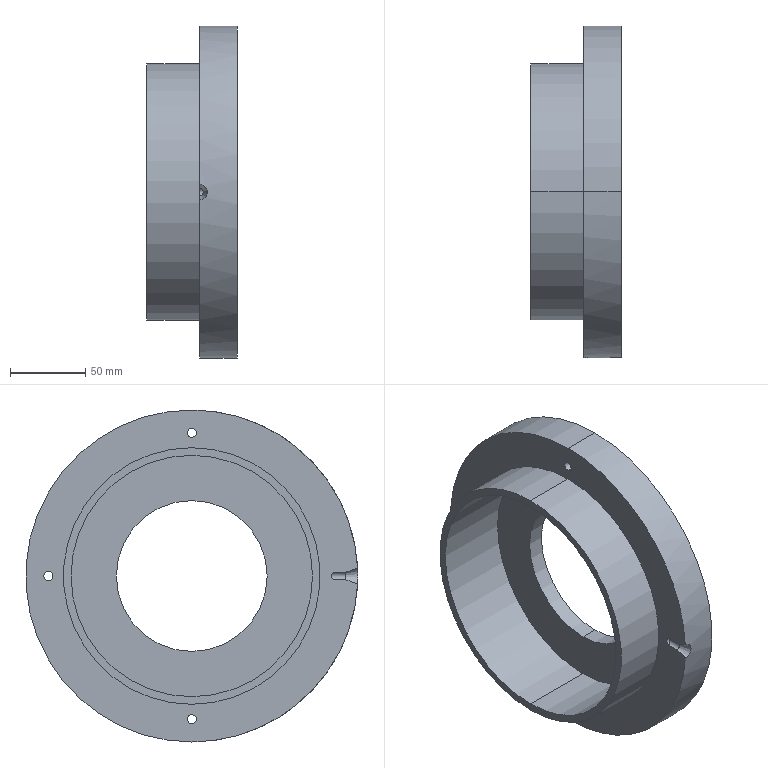Component | SolidWorks | EndCap-1 | 1 solid | 27 faces | box 60 x 220 x 220 mm | volume 670749 mm3 | cylinder 16 | cone 7 | plane 4 | commonest cylinder face diameters 6 x6 100 x2 160 x2 170 x2 220 x2 5 x2
STEP:
#1=COLOUR_RGB('',0.7922,0.8196,0.9333);
#2=FILL_AREA_STYLE_COLOUR('',#1);
#3=FILL_AREA_STYLE('',(#2));
#4=SURFACE_STYLE_FILL_AREA(#3);
#5=SURFACE_SIDE_STYLE('',(#4));
#6=SURFACE_STYLE_USAGE(.BOTH.,#5);
#7=PRESENTATION_STYLE_ASSIGNMENT((#6));
#8=CARTESIAN_POINT('',(-0.01969,3.74,0.1181));
#9=VERTEX_POINT('',#8);
#10=CARTESIAN_POINT('',(-0.01969,3.74,-0.1181));
#11=VERTEX_POINT('',#10);
#12=CARTESIAN_POINT('',(-0.01969,3.74,-0.));
#13=DIRECTION('',(1.,0.,-0.));
#14=DIRECTION('',(0.,0.,1.));
#15=AXIS2_PLACEMENT_3D('',#12,#13,#14);
#16=CIRCLE('',#15,0.1181);
#17=EDGE_CURVE('',#9,#11,#16,.T.);
#18=ORIENTED_EDGE('',*,*,#17,.F.);
#19=CARTESIAN_POINT('',(-0.,3.74,0.1378));
#20=VERTEX_POINT('',#19);
#21=CARTESIAN_POINT('',(-0.,3.74,0.1378));
#22=DIRECTION('',(0.7071,0.,0.7071));
#23=VECTOR('',#22,39.37);
#24=LINE('',#21,#23);
#25=EDGE_CURVE('',#9,#20,#24,.T.);
#26=ORIENTED_EDGE('',*,*,#25,.T.);
#27=CARTESIAN_POINT('',(-0.,3.74,-0.1378));
#28=VERTEX_POINT('',#27);
#29=CARTESIAN_POINT('',(-0.,3.74,-0.));
#30=DIRECTION('',(-1.,-0.,0.));
#31=DIRECTION('',(0.,0.,1.));
#32=AXIS2_PLACEMENT_3D('',#29,#30,#31);
#33=CIRCLE('',#32,0.1378);
#34=EDGE_CURVE('',#28,#20,#33,.T.);
#35=ORIENTED_EDGE('',*,*,#34,.F.);
#36=CARTESIAN_POINT('',(-0.,3.74,-0.1378));
#37=DIRECTION('',(0.7071,0.,-0.7071));
#38=VECTOR('',#37,39.37);
#39=LINE('',#36,#38);
#40=EDGE_CURVE('',#11,#28,#39,.T.);
#41=ORIENTED_EDGE('',*,*,#40,.F.);
#42=EDGE_LOOP('',(#18,#26,#35,#41));
#43=FACE_OUTER_BOUND('',#42,.T.);
#44=CARTESIAN_POINT('',(-0.,3.74,-0.));
#45=DIRECTION('',(1.,0.,-0.));
#46=DIRECTION('',(-0.,0.,-1.));
#47=AXIS2_PLACEMENT_3D('',#44,#45,#46);
#48=CONICAL_SURFACE('',#47,0.1378,0.7854);
#49=ADVANCED_FACE('',(#43),#48,.F.);
#50=CARTESIAN_POINT('',(-0.01969,-0.,-3.622));
#51=VERTEX_POINT('',#50);
#52=CARTESIAN_POINT('',(-0.01969,-0.,-3.858));
#53=VERTEX_POINT('',#52);
#54=CARTESIAN_POINT('',(-0.01969,-0.,-3.74));
#55=DIRECTION('',(1.,0.,-0.));
#56=DIRECTION('',(0.,0.,1.));
#57=AXIS2_PLACEMENT_3D('',#54,#55,#56);
#58=CIRCLE('',#57,0.1181);
#59=EDGE_CURVE('',#51,#53,#58,.T.);
#60=ORIENTED_EDGE('',*,*,#59,.F.);
#61=CARTESIAN_POINT('',(-0.,0.,-3.602));
#62=VERTEX_POINT('',#61);
#63=CARTESIAN_POINT('',(-0.,0.,-3.602));
#64=DIRECTION('',(0.7071,0.,0.7071));
#65=VECTOR('',#64,39.37);
#66=LINE('',#63,#65);
#67=EDGE_CURVE('',#51,#62,#66,.T.);
#68=ORIENTED_EDGE('',*,*,#67,.T.);
#69=CARTESIAN_POINT('',(-0.,0.,-3.878));
#70=VERTEX_POINT('',#69);
#71=CARTESIAN_POINT('',(-0.,0.,-3.74));
#72=DIRECTION('',(-1.,-0.,0.));
#73=DIRECTION('',(0.,0.,1.));
#74=AXIS2_PLACEMENT_3D('',#71,#72,#73);
#75=CIRCLE('',#74,0.1378);
#76=EDGE_CURVE('',#70,#62,#75,.T.);
#77=ORIENTED_EDGE('',*,*,#76,.F.);
#78=CARTESIAN_POINT('',(-0.,0.,-3.878));
#79=DIRECTION('',(0.7071,0.,-0.7071));
#80=VECTOR('',#79,39.37);
#81=LINE('',#78,#80);
#82=EDGE_CURVE('',#53,#70,#81,.T.);
#83=ORIENTED_EDGE('',*,*,#82,.F.);
#84=EDGE_LOOP('',(#60,#68,#77,#83));
#85=FACE_OUTER_BOUND('',#84,.T.);
#86=CARTESIAN_POINT('',(-0.,0.,-3.74));
#87=DIRECTION('',(1.,0.,-0.));
#88=DIRECTION('',(-0.,0.,-1.));
#89=AXIS2_PLACEMENT_3D('',#86,#87,#88);
#90=CONICAL_SURFACE('',#89,0.1378,0.7854);
#91=ADVANCED_FACE('',(#85),#90,.F.);
#92=CARTESIAN_POINT('',(-0.01969,-0.,3.858));
#93=VERTEX_POINT('',#92);
#94=CARTESIAN_POINT('',(-0.01969,-0.,3.622));
#95=VERTEX_POINT('',#94);
#96=CARTESIAN_POINT('',(-0.01969,-0.,3.74));
#97=DIRECTION('',(1.,0.,-0.));
#98=DIRECTION('',(0.,0.,1.));
#99=AXIS2_PLACEMENT_3D('',#96,#97,#98);
#100=CIRCLE('',#99,0.1181);
#101=EDGE_CURVE('',#93,#95,#100,.T.);
#102=ORIENTED_EDGE('',*,*,#101,.F.);
#103=CARTESIAN_POINT('',(0.,0.,3.878));
#104=VERTEX_POINT('',#103);
#105=CARTESIAN_POINT('',(0.,0.,3.878));
#106=DIRECTION('',(0.7071,0.,0.7071));
#107=VECTOR('',#106,39.37);
#108=LINE('',#105,#107);
#109=EDGE_CURVE('',#93,#104,#108,.T.);
#110=ORIENTED_EDGE('',*,*,#109,.T.);
#111=CARTESIAN_POINT('',(0.,0.,3.602));
#112=VERTEX_POINT('',#111);
#113=CARTESIAN_POINT('',(0.,0.,3.74));
#114=DIRECTION('',(-1.,-0.,0.));
#115=DIRECTION('',(0.,0.,1.));
#116=AXIS2_PLACEMENT_3D('',#113,#114,#115);
#117=CIRCLE('',#116,0.1378);
#118=EDGE_CURVE('',#112,#104,#117,.T.);
#119=ORIENTED_EDGE('',*,*,#118,.F.);
#120=CARTESIAN_POINT('',(0.,0.,3.602));
#121=DIRECTION('',(0.7071,0.,-0.7071));
#122=VECTOR('',#121,39.37);
#123=LINE('',#120,#122);
#124=EDGE_CURVE('',#95,#112,#123,.T.);
#125=ORIENTED_EDGE('',*,*,#124,.F.);
#126=EDGE_LOOP('',(#102,#110,#119,#125));
#127=FACE_OUTER_BOUND('',#126,.T.);
#128=CARTESIAN_POINT('',(0.,0.,3.74));
#129=DIRECTION('',(1.,0.,-0.));
#130=DIRECTION('',(-0.,0.,-1.));
#131=AXIS2_PLACEMENT_3D('',#128,#129,#130);
#132=CONICAL_SURFACE('',#131,0.1378,0.7854);
#133=ADVANCED_FACE('',(#127),#132,.F.);
#134=ORIENTED_EDGE('',*,*,#17,.T.);
#135=CARTESIAN_POINT('',(-0.9843,3.74,-0.1181));
#136=VERTEX_POINT('',#135);
#137=CARTESIAN_POINT('',(-0.,3.74,-0.1181));
#138=DIRECTION('',(-1.,-0.,0.));
#139=VECTOR('',#138,39.37);
#140=LINE('',#137,#139);
#141=EDGE_CURVE('',#11,#136,#140,.T.);
#142=ORIENTED_EDGE('',*,*,#141,.T.);
#143=CARTESIAN_POINT('',(-0.9843,3.74,0.1181));
#144=VERTEX_POINT('',#143);
#145=CARTESIAN_POINT('',(-0.9843,3.74,-0.));
#146=DIRECTION('',(-1.,-0.,0.));
#147=DIRECTION('',(0.,1.,-0.));
#148=AXIS2_PLACEMENT_3D('',#145,#146,#147);
#149=CIRCLE('',#148,0.1181);
#150=EDGE_CURVE('',#136,#144,#149,.T.);
#151=ORIENTED_EDGE('',*,*,#150,.T.);
#152=CARTESIAN_POINT('',(-0.,3.74,0.1181));
#153=DIRECTION('',(-1.,-0.,0.));
#154=VECTOR('',#153,39.37);
#155=LINE('',#152,#154);
#156=EDGE_CURVE('',#9,#144,#155,.T.);
#157=ORIENTED_EDGE('',*,*,#156,.F.);
#158=EDGE_LOOP('',(#134,#142,#151,#157));
#159=FACE_OUTER_BOUND('',#158,.T.);
#160=CARTESIAN_POINT('',(-0.,3.74,-0.));
#161=DIRECTION('',(-1.,-0.,0.));
#162=DIRECTION('',(0.,0.,1.));
#163=AXIS2_PLACEMENT_3D('',#160,#161,#162);
#164=CYLINDRICAL_SURFACE('',#163,0.1181);
#165=ADVANCED_FACE('',(#159),#164,.F.);
#166=ORIENTED_EDGE('',*,*,#59,.T.);
#167=CARTESIAN_POINT('',(-0.9843,-0.,-3.858));
#168=VERTEX_POINT('',#167);
#169=CARTESIAN_POINT('',(-0.,0.,-3.858));
#170=DIRECTION('',(-1.,-0.,0.));
#171=VECTOR('',#170,39.37);
#172=LINE('',#169,#171);
#173=EDGE_CURVE('',#53,#168,#172,.T.);
#174=ORIENTED_EDGE('',*,*,#173,.T.);
#175=CARTESIAN_POINT('',(-0.9843,-0.,-3.622));
#176=VERTEX_POINT('',#175);
#177=CARTESIAN_POINT('',(-0.9843,-0.,-3.74));
#178=DIRECTION('',(-1.,-0.,0.));
#179=DIRECTION('',(0.,0.,-1.));
#180=AXIS2_PLACEMENT_3D('',#177,#178,#179);
#181=CIRCLE('',#180,0.1181);
#182=EDGE_CURVE('',#168,#176,#181,.T.);
#183=ORIENTED_EDGE('',*,*,#182,.T.);
#184=CARTESIAN_POINT('',(-0.,0.,-3.622));
#185=DIRECTION('',(-1.,-0.,0.));
#186=VECTOR('',#185,39.37);
#187=LINE('',#184,#186);
#188=EDGE_CURVE('',#51,#176,#187,.T.);
#189=ORIENTED_EDGE('',*,*,#188,.F.);
#190=EDGE_LOOP('',(#166,#174,#183,#189));
#191=FACE_OUTER_BOUND('',#190,.T.);
#192=CARTESIAN_POINT('',(-0.,0.,-3.74));
#193=DIRECTION('',(-1.,-0.,0.));
#194=DIRECTION('',(0.,0.,1.));
#195=AXIS2_PLACEMENT_3D('',#192,#193,#194);
#196=CYLINDRICAL_SURFACE('',#195,0.1181);
#197=ADVANCED_FACE('',(#191),#196,.F.);
#198=ORIENTED_EDGE('',*,*,#101,.T.);
#199=CARTESIAN_POINT('',(-0.9843,-0.,3.622));
#200=VERTEX_POINT('',#199);
#201=CARTESIAN_POINT('',(0.,0.,3.622));
#202=DIRECTION('',(-1.,-0.,0.));
#203=VECTOR('',#202,39.37);
#204=LINE('',#201,#203);
#205=EDGE_CURVE('',#95,#200,#204,.T.);
#206=ORIENTED_EDGE('',*,*,#205,.T.);
#207=CARTESIAN_POINT('',(-0.9843,-0.,3.858));
#208=VERTEX_POINT('',#207);
#209=CARTESIAN_POINT('',(-0.9843,-0.,3.74));
#210=DIRECTION('',(-1.,-0.,0.));
#211=DIRECTION('',(0.,0.,1.));
#212=AXIS2_PLACEMENT_3D('',#209,#210,#211);
#213=CIRCLE('',#212,0.1181);
#214=EDGE_CURVE('',#200,#208,#213,.T.);
#215=ORIENTED_EDGE('',*,*,#214,.T.);
#216=CARTESIAN_POINT('',(0.,0.,3.858));
#217=DIRECTION('',(-1.,-0.,0.));
#218=VECTOR('',#217,39.37);
#219=LINE('',#216,#218);
#220=EDGE_CURVE('',#93,#208,#219,.T.);
#221=ORIENTED_EDGE('',*,*,#220,.F.);
#222=EDGE_LOOP('',(#198,#206,#215,#221));
#223=FACE_OUTER_BOUND('',#222,.T.);
#224=CARTESIAN_POINT('',(0.,0.,3.74));
#225=DIRECTION('',(-1.,-0.,0.));
#226=DIRECTION('',(0.,0.,1.));
#227=AXIS2_PLACEMENT_3D('',#224,#225,#226);
#228=CYLINDRICAL_SURFACE('',#227,0.1181);
#229=ADVANCED_FACE('',(#223),#228,.F.);
#230=CARTESIAN_POINT('',(-0.,0.,-1.969));
#231=VERTEX_POINT('',#230);
#232=CARTESIAN_POINT('',(0.,0.,1.969));
#233=VERTEX_POINT('',#232);
#234=CARTESIAN_POINT('',(0.,0.,0.));
#235=DIRECTION('',(-1.,-0.,0.));
#236=DIRECTION('',(0.,0.,1.));
#237=AXIS2_PLACEMENT_3D('',#234,#235,#236);
#238=CIRCLE('',#237,1.969);
#239=EDGE_CURVE('',#231,#233,#238,.T.);
#240=ORIENTED_EDGE('',*,*,#239,.F.);
#241=CARTESIAN_POINT('',(-0.4331,0.,-1.969));
#242=VERTEX_POINT('',#241);
#243=CARTESIAN_POINT('',(-0.,0.,-1.969));
#244=DIRECTION('',(-1.,-0.,0.));
#245=VECTOR('',#244,39.37);
#246=LINE('',#243,#245);
#247=EDGE_CURVE('',#231,#242,#246,.T.);
#248=ORIENTED_EDGE('',*,*,#247,.T.);
#249=CARTESIAN_POINT('',(-0.4331,-0.,1.969));
#250=VERTEX_POINT('',#249);
#251=CARTESIAN_POINT('',(-0.4331,-0.,0.));
#252=DIRECTION('',(-1.,-0.,0.));
#253=DIRECTION('',(0.,0.,1.));
#254=AXIS2_PLACEMENT_3D('',#251,#252,#253);
#255=CIRCLE('',#254,1.969);
#256=EDGE_CURVE('',#242,#250,#255,.T.);
#257=ORIENTED_EDGE('',*,*,#256,.T.);
#258=CARTESIAN_POINT('',(0.,0.,1.969));
#259=DIRECTION('',(-1.,-0.,0.));
#260=VECTOR('',#259,39.37);
#261=LINE('',#258,#260);
#262=EDGE_CURVE('',#233,#250,#261,.T.);
#263=ORIENTED_EDGE('',*,*,#262,.F.);
#264=EDGE_LOOP('',(#240,#248,#257,#263));
#265=FACE_OUTER_BOUND('',#264,.T.);
#266=CARTESIAN_POINT('',(0.,0.,0.));
#267=DIRECTION('',(-1.,-0.,0.));
#268=DIRECTION('',(0.,0.,1.));
#269=AXIS2_PLACEMENT_3D('',#266,#267,#268);
#270=CYLINDRICAL_SURFACE('',#269,1.969);
#271=ADVANCED_FACE('',(#265),#270,.F.);
#272=CARTESIAN_POINT('',(-0.4331,-0.,-3.15));
#273=VERTEX_POINT('',#272);
#274=CARTESIAN_POINT('',(-0.4331,-0.,3.15));
#275=VERTEX_POINT('',#274);
#276=CARTESIAN_POINT('',(-0.4331,-0.,0.));
#277=DIRECTION('',(-1.,-0.,0.));
#278=DIRECTION('',(0.,0.,1.));
#279=AXIS2_PLACEMENT_3D('',#276,#277,#278);
#280=CIRCLE('',#279,3.15);
#281=EDGE_CURVE('',#273,#275,#280,.T.);
#282=ORIENTED_EDGE('',*,*,#281,.F.);
#283=CARTESIAN_POINT('',(-2.362,-0.,-3.15));
#284=VERTEX_POINT('',#283);
#285=CARTESIAN_POINT('',(-0.4331,0.,-3.15));
#286=DIRECTION('',(-1.,-0.,0.));
#287=VECTOR('',#286,39.37);
#288=LINE('',#285,#287);
#289=EDGE_CURVE('',#273,#284,#288,.T.);
#290=ORIENTED_EDGE('',*,*,#289,.T.);
#291=CARTESIAN_POINT('',(-2.362,-0.,3.15));
#292=VERTEX_POINT('',#291);
#293=CARTESIAN_POINT('',(-2.362,-0.,0.));
#294=DIRECTION('',(-1.,-0.,0.));
#295=DIRECTION('',(0.,0.,1.));
#296=AXIS2_PLACEMENT_3D('',#293,#294,#295);
#297=CIRCLE('',#296,3.15);
#298=EDGE_CURVE('',#284,#292,#297,.T.);
#299=ORIENTED_EDGE('',*,*,#298,.T.);
#300=CARTESIAN_POINT('',(-0.4331,-0.,3.15));
#301=DIRECTION('',(-1.,-0.,0.));
#302=VECTOR('',#301,39.37);
#303=LINE('',#300,#302);
#304=EDGE_CURVE('',#275,#292,#303,.T.);
#305=ORIENTED_EDGE('',*,*,#304,.F.);
#306=EDGE_LOOP('',(#282,#290,#299,#305));
#307=FACE_OUTER_BOUND('',#306,.T.);
#308=CARTESIAN_POINT('',(-0.4331,-0.,0.));
#309=DIRECTION('',(-1.,-0.,0.));
#310=DIRECTION('',(0.,0.,1.));
#311=AXIS2_PLACEMENT_3D('',#308,#309,#310);
#312=CYLINDRICAL_SURFACE('',#311,3.15);
#313=ADVANCED_FACE('',(#307),#312,.F.);
#314=CARTESIAN_POINT('',(-2.362,-0.,3.346));
#315=VERTEX_POINT('',#314);
#316=CARTESIAN_POINT('',(-2.362,-0.,-3.346));
#317=VERTEX_POINT('',#316);
#318=CARTESIAN_POINT('',(-2.362,-0.,0.));
#319=DIRECTION('',(-1.,-0.,0.));
#320=DIRECTION('',(0.,0.,1.));
#321=AXIS2_PLACEMENT_3D('',#318,#319,#320);
#322=CIRCLE('',#321,3.346);
#323=EDGE_CURVE('',#315,#317,#322,.T.);
#324=ORIENTED_EDGE('',*,*,#323,.F.);
#325=CARTESIAN_POINT('',(-0.9843,-0.,3.346));
#326=VERTEX_POINT('',#325);
#327=CARTESIAN_POINT('',(-2.362,-0.,3.346));
#328=DIRECTION('',(1.,0.,-0.));
#329=VECTOR('',#328,39.37);
#330=LINE('',#327,#329);
#331=EDGE_CURVE('',#315,#326,#330,.T.);
#332=ORIENTED_EDGE('',*,*,#331,.T.);
#333=CARTESIAN_POINT('',(-0.9843,-0.,-3.346));
#334=VERTEX_POINT('',#333);
#335=CARTESIAN_POINT('',(-0.9843,-0.,0.));
#336=DIRECTION('',(-1.,-0.,0.));
#337=DIRECTION('',(0.,0.,1.));
#338=AXIS2_PLACEMENT_3D('',#335,#336,#337);
#339=CIRCLE('',#338,3.346);
#340=EDGE_CURVE('',#326,#334,#339,.T.);
#341=ORIENTED_EDGE('',*,*,#340,.T.);
#342=CARTESIAN_POINT('',(-2.362,-0.,-3.346));
#343=DIRECTION('',(1.,0.,-0.));
#344=VECTOR('',#343,39.37);
#345=LINE('',#342,#344);
#346=EDGE_CURVE('',#317,#334,#345,.T.);
#347=ORIENTED_EDGE('',*,*,#346,.F.);
#348=EDGE_LOOP('',(#324,#332,#341,#347));
#349=FACE_OUTER_BOUND('',#348,.T.);
#350=CARTESIAN_POINT('',(-2.362,-0.,0.));
#351=DIRECTION('',(1.,0.,-0.));
#352=DIRECTION('',(0.,0.,-1.));
#353=AXIS2_PLACEMENT_3D('',#350,#351,#352);
#354=CYLINDRICAL_SURFACE('',#353,3.346);
#355=ADVANCED_FACE('',(#349),#354,.T.);
#356=CARTESIAN_POINT('',(-0.9843,0.,4.331));
#357=VERTEX_POINT('',#356);
#358=CARTESIAN_POINT('',(-0.9843,-0.,-4.331));
#359=VERTEX_POINT('',#358);
#360=CARTESIAN_POINT('',(-0.9843,-0.,0.));
#361=DIRECTION('',(-1.,-0.,0.));
#362=DIRECTION('',(0.,0.,1.));
#363=AXIS2_PLACEMENT_3D('',#360,#361,#362);
#364=CIRCLE('',#363,4.331);
#365=EDGE_CURVE('',#357,#359,#364,.T.);
#366=ORIENTED_EDGE('',*,*,#365,.F.);
#367=CARTESIAN_POINT('',(0.,0.,4.331));
#368=VERTEX_POINT('',#367);
#369=CARTESIAN_POINT('',(-0.9843,0.,4.331));
#370=DIRECTION('',(1.,0.,-0.));
#371=VECTOR('',#370,39.37);
#372=LINE('',#369,#371);
#373=EDGE_CURVE('',#357,#368,#372,.T.);
#374=ORIENTED_EDGE('',*,*,#373,.T.);
#375=CARTESIAN_POINT('',(-0.,-0.,-4.331));
#376=VERTEX_POINT('',#375);
#377=CARTESIAN_POINT('',(0.,0.,0.));
#378=DIRECTION('',(-1.,-0.,0.));
#379=DIRECTION('',(0.,0.,1.));
#380=AXIS2_PLACEMENT_3D('',#377,#378,#379);
#381=CIRCLE('',#380,4.331);
#382=EDGE_CURVE('',#368,#376,#381,.T.);
#383=ORIENTED_EDGE('',*,*,#382,.T.);
#384=CARTESIAN_POINT('',(-0.9843,-0.,-4.331));
#385=DIRECTION('',(1.,0.,-0.));
#386=VECTOR('',#385,39.37);
#387=LINE('',#384,#386);
#388=EDGE_CURVE('',#359,#376,#387,.T.);
#389=ORIENTED_EDGE('',*,*,#388,.F.);
#390=EDGE_LOOP('',(#366,#374,#383,#389));
#391=FACE_OUTER_BOUND('',#390,.T.);
#392=CARTESIAN_POINT('',(-0.9843,-0.,0.));
#393=DIRECTION('',(1.,0.,-0.));
#394=DIRECTION('',(0.,0.,-1.));
#395=AXIS2_PLACEMENT_3D('',#392,#393,#394);
#396=CYLINDRICAL_SURFACE('',#395,4.331);
#397=ADVANCED_FACE('',(#391),#396,.T.);
#398=ORIENTED_EDGE('',*,*,#373,.F.);
#399=CARTESIAN_POINT('',(-0.9843,-4.326,0.2074));
#400=VERTEX_POINT('',#399);
#401=CARTESIAN_POINT('',(-0.9843,-0.,0.));
#402=DIRECTION('',(-1.,-0.,0.));
#403=DIRECTION('',(0.,0.,1.));
#404=AXIS2_PLACEMENT_3D('',#401,#402,#403);
#405=CIRCLE('',#404,4.331);
#406=EDGE_CURVE('',#400,#357,#405,.T.);
#407=ORIENTED_EDGE('',*,*,#406,.F.);
#408=CARTESIAN_POINT('',(-0.9843,-4.326,-0.2074));
#409=VERTEX_POINT('',#408);
#410=CARTESIAN_POINT('',(-0.9843,-4.326,0.2074));
#411=CARTESIAN_POINT('',(-0.9705,-4.326,0.2074));
#412=CARTESIAN_POINT('',(-0.957,-4.326,0.206));
#413=CARTESIAN_POINT('',(-0.9305,-4.326,0.2008));
#414=CARTESIAN_POINT('',(-0.9174,-4.326,0.197));
#415=CARTESIAN_POINT('',(-0.892,-4.327,0.1866));
#416=CARTESIAN_POINT('',(-0.8799,-4.327,0.1802));
#417=CARTESIAN_POINT('',(-0.8629,-4.327,0.169));
#418=CARTESIAN_POINT('',(-0.8574,-4.328,0.165));
#419=CARTESIAN_POINT('',(-0.8468,-4.328,0.1564));
#420=CARTESIAN_POINT('',(-0.8416,-4.328,0.1518));
#421=CARTESIAN_POINT('',(-0.8271,-4.329,0.1375));
#422=CARTESIAN_POINT('',(-0.8184,-4.329,0.127));
#423=CARTESIAN_POINT('',(-0.8031,-4.329,0.1045));
#424=CARTESIAN_POINT('',(-0.7965,-4.33,0.09231));
#425=CARTESIAN_POINT('',(-0.786,-4.33,0.06727));
#426=CARTESIAN_POINT('',(-0.782,-4.33,0.0543));
#427=CARTESIAN_POINT('',(-0.7765,-4.331,0.02743));
#428=CARTESIAN_POINT('',(-0.7751,-4.331,0.01377));
#429=CARTESIAN_POINT('',(-0.7751,-4.331,-0.006587));
#430=CARTESIAN_POINT('',(-0.7754,-4.331,-0.01337));
#431=CARTESIAN_POINT('',(-0.7768,-4.331,-0.02695));
#432=CARTESIAN_POINT('',(-0.7778,-4.331,-0.03378));
#433=CARTESIAN_POINT('',(-0.7818,-4.33,-0.05392));
#434=CARTESIAN_POINT('',(-0.7858,-4.33,-0.06689));
#435=CARTESIAN_POINT('',(-0.7963,-4.33,-0.09198));
#436=CARTESIAN_POINT('',(-0.8029,-4.329,-0.1042));
#437=CARTESIAN_POINT('',(-0.8182,-4.329,-0.1267));
#438=CARTESIAN_POINT('',(-0.8268,-4.329,-0.1372));
#439=CARTESIAN_POINT('',(-0.8414,-4.328,-0.1516));
#440=CARTESIAN_POINT('',(-0.8465,-4.328,-0.1562));
#441=CARTESIAN_POINT('',(-0.8572,-4.328,-0.1648));
#442=CARTESIAN_POINT('',(-0.8626,-4.327,-0.1688));
#443=CARTESIAN_POINT('',(-0.8796,-4.327,-0.18));
#444=CARTESIAN_POINT('',(-0.8917,-4.327,-0.1864));
#445=CARTESIAN_POINT('',(-0.9171,-4.326,-0.1969));
#446=CARTESIAN_POINT('',(-0.9301,-4.326,-0.2008));
#447=CARTESIAN_POINT('',(-0.9568,-4.326,-0.206));
#448=CARTESIAN_POINT('',(-0.9705,-4.326,-0.2074));
#449=CARTESIAN_POINT('',(-0.9843,-4.326,-0.2074));
#450=B_SPLINE_CURVE_WITH_KNOTS('',3,(#410,#411,#412,#413,#414,#415,#416,#417,#418,#419,#420,#421,#422,#423,#424,#425,#426,#427,#428,#429,#430,#431,#432,#433,#434,#435,#436,#437,#438,#439,#440,#441,#442,#443,#444,#445,#446,#447,#448,#449),.UNSPECIFIED.,.F.,.F.,(4,2,2,2,2,2,2,2,2,2,2,2,2,2,2,2,2,2,2,4),(0.0000002,0.00103,0.00206,0.00309,0.003605,0.00412,0.00515,0.00618,0.00721,0.00824,0.008755,0.00927,0.0103,0.01133,0.01236,0.01288,0.01339,0.01442,0.01545,0.01648),.UNSPECIFIED.);
#451=EDGE_CURVE('',#400,#409,#450,.T.);
#452=ORIENTED_EDGE('',*,*,#451,.T.);
#453=CARTESIAN_POINT('',(-0.9843,-0.,0.));
#454=DIRECTION('',(-1.,-0.,0.));
#455=DIRECTION('',(0.,0.,1.));
#456=AXIS2_PLACEMENT_3D('',#453,#454,#455);
#457=CIRCLE('',#456,4.331);
#458=EDGE_CURVE('',#359,#409,#457,.T.);
#459=ORIENTED_EDGE('',*,*,#458,.F.);
#460=ORIENTED_EDGE('',*,*,#388,.T.);
#461=CARTESIAN_POINT('',(0.,0.,0.));
#462=DIRECTION('',(-1.,-0.,0.));
#463=DIRECTION('',(0.,0.,1.));
#464=AXIS2_PLACEMENT_3D('',#461,#462,#463);
#465=CIRCLE('',#464,4.331);
#466=EDGE_CURVE('',#376,#368,#465,.T.);
#467=ORIENTED_EDGE('',*,*,#466,.T.);
#468=EDGE_LOOP('',(#398,#407,#452,#459,#460,#467));
#469=FACE_OUTER_BOUND('',#468,.T.);
#470=CARTESIAN_POINT('',(-0.9843,-0.,0.));
#471=DIRECTION('',(1.,0.,-0.));
#472=DIRECTION('',(0.,0.,-1.));
#473=AXIS2_PLACEMENT_3D('',#470,#471,#472);
#474=CYLINDRICAL_SURFACE('',#473,4.331);
#475=ADVANCED_FACE('',(#469),#474,.T.);
#476=CARTESIAN_POINT('',(-0.9843,-4.018,-0.09843));
#477=VERTEX_POINT('',#476);
#478=CARTESIAN_POINT('',(-0.9843,-3.74,0.));
#479=DIRECTION('',(0.,-0.9426,-0.3338));
#480=VECTOR('',#479,39.37);
#481=LINE('',#478,#480);
#482=EDGE_CURVE('',#477,#409,#481,.T.);
#483=ORIENTED_EDGE('',*,*,#482,.F.);
#484=CARTESIAN_POINT('',(-0.9843,-3.74,-0.09843));
#485=VERTEX_POINT('',#484);
#486=CARTESIAN_POINT('',(-0.9843,-5.118,-0.09843));
#487=DIRECTION('',(0.,1.,-0.));
#488=VECTOR('',#487,39.37);
#489=LINE('',#486,#488);
#490=EDGE_CURVE('',#477,#485,#489,.T.);
#491=ORIENTED_EDGE('',*,*,#490,.T.);
#492=CARTESIAN_POINT('',(-0.9843,-3.74,0.09843));
#493=VERTEX_POINT('',#492);
#494=CARTESIAN_POINT('',(-0.9843,-3.74,0.));
#495=DIRECTION('',(1.,0.,-0.));
#496=DIRECTION('',(0.,0.,1.));
#497=AXIS2_PLACEMENT_3D('',#494,#495,#496);
#498=CIRCLE('',#497,0.09843);
#499=EDGE_CURVE('',#485,#493,#498,.T.);
#500=ORIENTED_EDGE('',*,*,#499,.T.);
#501=CARTESIAN_POINT('',(-0.9843,-4.018,0.09843));
#502=VERTEX_POINT('',#501);
#503=CARTESIAN_POINT('',(-0.9843,-5.118,0.09843));
#504=DIRECTION('',(-0.,-1.,0.));
#505=VECTOR('',#504,39.37);
#506=LINE('',#503,#505);
#507=EDGE_CURVE('',#493,#502,#506,.T.);
#508=ORIENTED_EDGE('',*,*,#507,.T.);
#509=CARTESIAN_POINT('',(-0.9843,-3.74,0.));
#510=DIRECTION('',(-0.,0.9426,-0.3338));
#511=VECTOR('',#510,39.37);
#512=LINE('',#509,#511);
#513=EDGE_CURVE('',#400,#502,#512,.T.);
#514=ORIENTED_EDGE('',*,*,#513,.F.);
#515=ORIENTED_EDGE('',*,*,#406,.T.);
#516=ORIENTED_EDGE('',*,*,#365,.T.);
#517=ORIENTED_EDGE('',*,*,#458,.T.);
#518=EDGE_LOOP('',(#483,#491,#500,#508,#514,#515,#516,#517));
#519=FACE_OUTER_BOUND('',#518,.T.);
#520=CARTESIAN_POINT('',(-0.9843,3.74,-0.));
#521=DIRECTION('',(-1.,-0.,0.));
#522=DIRECTION('',(0.,1.,-0.));
#523=AXIS2_PLACEMENT_3D('',#520,#521,#522);
#524=CIRCLE('',#523,0.1181);
#525=EDGE_CURVE('',#144,#136,#524,.T.);
#526=ORIENTED_EDGE('',*,*,#525,.F.);
#527=ORIENTED_EDGE('',*,*,#150,.F.);
#528=EDGE_LOOP('',(#526,#527));
#529=FACE_BOUND('',#528,.T.);
#530=CARTESIAN_POINT('',(-0.9843,-0.,-3.74));
#531=DIRECTION('',(-1.,-0.,0.));
#532=DIRECTION('',(0.,0.,-1.));
#533=AXIS2_PLACEMENT_3D('',#530,#531,#532);
#534=CIRCLE('',#533,0.1181);
#535=EDGE_CURVE('',#176,#168,#534,.T.);
#536=ORIENTED_EDGE('',*,*,#535,.F.);
#537=ORIENTED_EDGE('',*,*,#182,.F.);
#538=EDGE_LOOP('',(#536,#537));
#539=FACE_BOUND('',#538,.T.);
#540=CARTESIAN_POINT('',(-0.9843,-0.,3.74));
#541=DIRECTION('',(-1.,-0.,0.));
#542=DIRECTION('',(0.,0.,1.));
#543=AXIS2_PLACEMENT_3D('',#540,#541,#542);
#544=CIRCLE('',#543,0.1181);
#545=EDGE_CURVE('',#208,#200,#544,.T.);
#546=ORIENTED_EDGE('',*,*,#545,.F.);
#547=ORIENTED_EDGE('',*,*,#214,.F.);
#548=EDGE_LOOP('',(#546,#547));
#549=FACE_BOUND('',#548,.T.);
#550=CARTESIAN_POINT('',(-0.9843,-0.,0.));
#551=DIRECTION('',(-1.,-0.,0.));
#552=DIRECTION('',(0.,0.,1.));
#553=AXIS2_PLACEMENT_3D('',#550,#551,#552);
#554=CIRCLE('',#553,3.346);
#555=EDGE_CURVE('',#334,#326,#554,.T.);
#556=ORIENTED_EDGE('',*,*,#555,.F.);
#557=ORIENTED_EDGE('',*,*,#340,.F.);
#558=EDGE_LOOP('',(#556,#557));
#559=FACE_BOUND('',#558,.T.);
#560=CARTESIAN_POINT('',(-0.9843,-0.,0.));
#561=DIRECTION('',(-1.,-0.,0.));
#562=DIRECTION('',(0.,0.,1.));
#563=AXIS2_PLACEMENT_3D('',#560,#561,#562);
#564=PLANE('',#563);
#565=ADVANCED_FACE('',(#519,#529,#539,#549,#559),#564,.T.);
#566=ORIENTED_EDGE('',*,*,#118,.T.);
#567=CARTESIAN_POINT('',(0.,0.,3.74));
#568=DIRECTION('',(-1.,-0.,0.));
#569=DIRECTION('',(0.,0.,1.));
#570=AXIS2_PLACEMENT_3D('',#567,#568,#569);
#571=CIRCLE('',#570,0.1378);
#572=EDGE_CURVE('',#104,#112,#571,.T.);
#573=ORIENTED_EDGE('',*,*,#572,.T.);
#574=EDGE_LOOP('',(#566,#573));
#575=FACE_BOUND('',#574,.T.);
#576=ORIENTED_EDGE('',*,*,#76,.T.);
#577=CARTESIAN_POINT('',(-0.,0.,-3.74));
#578=DIRECTION('',(-1.,-0.,0.));
#579=DIRECTION('',(0.,0.,1.));
#580=AXIS2_PLACEMENT_3D('',#577,#578,#579);
#581=CIRCLE('',#580,0.1378);
#582=EDGE_CURVE('',#62,#70,#581,.T.);
#583=ORIENTED_EDGE('',*,*,#582,.T.);
#584=EDGE_LOOP('',(#576,#583));
#585=FACE_BOUND('',#584,.T.);
#586=ORIENTED_EDGE('',*,*,#34,.T.);
#587=CARTESIAN_POINT('',(-0.,3.74,-0.));
#588=DIRECTION('',(-1.,-0.,0.));
#589=DIRECTION('',(0.,0.,1.));
#590=AXIS2_PLACEMENT_3D('',#587,#588,#589);
#591=CIRCLE('',#590,0.1378);
#592=EDGE_CURVE('',#20,#28,#591,.T.);
#593=ORIENTED_EDGE('',*,*,#592,.T.);
#594=EDGE_LOOP('',(#586,#593));
#595=FACE_BOUND('',#594,.T.);
#596=CARTESIAN_POINT('',(0.,0.,0.));
#597=DIRECTION('',(-1.,-0.,0.));
#598=DIRECTION('',(0.,0.,1.));
#599=AXIS2_PLACEMENT_3D('',#596,#597,#598);
#600=CIRCLE('',#599,1.969);
#601=EDGE_CURVE('',#233,#231,#600,.T.);
#602=ORIENTED_EDGE('',*,*,#601,.T.);
#603=ORIENTED_EDGE('',*,*,#239,.T.);
#604=EDGE_LOOP('',(#602,#603));
#605=FACE_BOUND('',#604,.T.);
#606=ORIENTED_EDGE('',*,*,#466,.F.);
#607=ORIENTED_EDGE('',*,*,#382,.F.);
#608=EDGE_LOOP('',(#606,#607));
#609=FACE_OUTER_BOUND('',#608,.T.);
#610=CARTESIAN_POINT('',(0.,0.,0.));
#611=DIRECTION('',(-1.,-0.,0.));
#612=DIRECTION('',(0.,0.,1.));
#613=AXIS2_PLACEMENT_3D('',#610,#611,#612);
#614=PLANE('',#613);
#615=ADVANCED_FACE('',(#575,#585,#595,#605,#609),#614,.F.);
#616=ORIENTED_EDGE('',*,*,#331,.F.);
#617=CARTESIAN_POINT('',(-2.362,-0.,0.));
#618=DIRECTION('',(-1.,-0.,0.));
#619=DIRECTION('',(0.,0.,1.));
#620=AXIS2_PLACEMENT_3D('',#617,#618,#619);
#621=CIRCLE('',#620,3.346);
#622=EDGE_CURVE('',#317,#315,#621,.T.);
#623=ORIENTED_EDGE('',*,*,#622,.F.);
#624=ORIENTED_EDGE('',*,*,#346,.T.);
#625=ORIENTED_EDGE('',*,*,#555,.T.);
#626=EDGE_LOOP('',(#616,#623,#624,#625));
#627=FACE_OUTER_BOUND('',#626,.T.);
#628=CARTESIAN_POINT('',(-2.362,-0.,0.));
#629=DIRECTION('',(1.,0.,-0.));
#630=DIRECTION('',(0.,0.,-1.));
#631=AXIS2_PLACEMENT_3D('',#628,#629,#630);
#632=CYLINDRICAL_SURFACE('',#631,3.346);
#633=ADVANCED_FACE('',(#627),#632,.T.);
#634=CARTESIAN_POINT('',(-2.362,-0.,0.));
#635=DIRECTION('',(-1.,-0.,0.));
#636=DIRECTION('',(0.,0.,1.));
#637=AXIS2_PLACEMENT_3D('',#634,#635,#636);
#638=CIRCLE('',#637,3.15);
#639=EDGE_CURVE('',#292,#284,#638,.T.);
#640=ORIENTED_EDGE('',*,*,#639,.F.);
#641=ORIENTED_EDGE('',*,*,#298,.F.);
#642=EDGE_LOOP('',(#640,#641));
#643=FACE_BOUND('',#642,.T.);
#644=ORIENTED_EDGE('',*,*,#622,.T.);
#645=ORIENTED_EDGE('',*,*,#323,.T.);
#646=EDGE_LOOP('',(#644,#645));
#647=FACE_OUTER_BOUND('',#646,.T.);
#648=CARTESIAN_POINT('',(-2.362,-0.,0.));
#649=DIRECTION('',(-1.,-0.,0.));
#650=DIRECTION('',(0.,0.,1.));
#651=AXIS2_PLACEMENT_3D('',#648,#649,#650);
#652=PLANE('',#651);
#653=ADVANCED_FACE('',(#643,#647),#652,.T.);
#654=ORIENTED_EDGE('',*,*,#289,.F.);
#655=CARTESIAN_POINT('',(-0.4331,-0.,0.));
#656=DIRECTION('',(-1.,-0.,0.));
#657=DIRECTION('',(0.,0.,1.));
#658=AXIS2_PLACEMENT_3D('',#655,#656,#657);
#659=CIRCLE('',#658,3.15);
#660=EDGE_CURVE('',#275,#273,#659,.T.);
#661=ORIENTED_EDGE('',*,*,#660,.F.);
#662=ORIENTED_EDGE('',*,*,#304,.T.);
#663=ORIENTED_EDGE('',*,*,#639,.T.);
#664=EDGE_LOOP('',(#654,#661,#662,#663));
#665=FACE_OUTER_BOUND('',#664,.T.);
#666=CARTESIAN_POINT('',(-0.4331,-0.,0.));
#667=DIRECTION('',(-1.,-0.,0.));
#668=DIRECTION('',(0.,0.,1.));
#669=AXIS2_PLACEMENT_3D('',#666,#667,#668);
#670=CYLINDRICAL_SURFACE('',#669,3.15);
#671=ADVANCED_FACE('',(#665),#670,.F.);
#672=CARTESIAN_POINT('',(-0.4331,-0.,0.));
#673=DIRECTION('',(-1.,-0.,0.));
#674=DIRECTION('',(0.,0.,1.));
#675=AXIS2_PLACEMENT_3D('',#672,#673,#674);
#676=CIRCLE('',#675,1.969);
#677=EDGE_CURVE('',#250,#242,#676,.T.);
#678=ORIENTED_EDGE('',*,*,#677,.F.);
#679=ORIENTED_EDGE('',*,*,#256,.F.);
#680=EDGE_LOOP('',(#678,#679));
#681=FACE_BOUND('',#680,.T.);
#682=ORIENTED_EDGE('',*,*,#660,.T.);
#683=ORIENTED_EDGE('',*,*,#281,.T.);
#684=EDGE_LOOP('',(#682,#683));
#685=FACE_OUTER_BOUND('',#684,.T.);
#686=CARTESIAN_POINT('',(-0.4331,-0.,0.));
#687=DIRECTION('',(-1.,-0.,0.));
#688=DIRECTION('',(0.,0.,1.));
#689=AXIS2_PLACEMENT_3D('',#686,#687,#688);
#690=PLANE('',#689);
#691=ADVANCED_FACE('',(#681,#685),#690,.T.);
#692=ORIENTED_EDGE('',*,*,#247,.F.);
#693=ORIENTED_EDGE('',*,*,#601,.F.);
#694=ORIENTED_EDGE('',*,*,#262,.T.);
#695=ORIENTED_EDGE('',*,*,#677,.T.);
#696=EDGE_LOOP('',(#692,#693,#694,#695));
#697=FACE_OUTER_BOUND('',#696,.T.);
#698=CARTESIAN_POINT('',(0.,0.,0.));
#699=DIRECTION('',(-1.,-0.,0.));
#700=DIRECTION('',(0.,0.,1.));
#701=AXIS2_PLACEMENT_3D('',#698,#699,#700);
#702=CYLINDRICAL_SURFACE('',#701,1.969);
#703=ADVANCED_FACE('',(#697),#702,.F.);
#704=ORIENTED_EDGE('',*,*,#205,.F.);
#705=CARTESIAN_POINT('',(-0.01969,-0.,3.74));
#706=DIRECTION('',(1.,0.,-0.));
#707=DIRECTION('',(0.,0.,1.));
#708=AXIS2_PLACEMENT_3D('',#705,#706,#707);
#709=CIRCLE('',#708,0.1181);
#710=EDGE_CURVE('',#95,#93,#709,.T.);
#711=ORIENTED_EDGE('',*,*,#710,.T.);
#712=ORIENTED_EDGE('',*,*,#220,.T.);
#713=ORIENTED_EDGE('',*,*,#545,.T.);
#714=EDGE_LOOP('',(#704,#711,#712,#713));
#715=FACE_OUTER_BOUND('',#714,.T.);
#716=CARTESIAN_POINT('',(0.,0.,3.74));
#717=DIRECTION('',(-1.,-0.,0.));
#718=DIRECTION('',(0.,0.,1.));
#719=AXIS2_PLACEMENT_3D('',#716,#717,#718);
#720=CYLINDRICAL_SURFACE('',#719,0.1181);
#721=ADVANCED_FACE('',(#715),#720,.F.);
#722=ORIENTED_EDGE('',*,*,#173,.F.);
#723=CARTESIAN_POINT('',(-0.01969,-0.,-3.74));
#724=DIRECTION('',(1.,0.,-0.));
#725=DIRECTION('',(0.,0.,1.));
#726=AXIS2_PLACEMENT_3D('',#723,#724,#725);
#727=CIRCLE('',#726,0.1181);
#728=EDGE_CURVE('',#53,#51,#727,.T.);
#729=ORIENTED_EDGE('',*,*,#728,.T.);
#730=ORIENTED_EDGE('',*,*,#188,.T.);
#731=ORIENTED_EDGE('',*,*,#535,.T.);
#732=EDGE_LOOP('',(#722,#729,#730,#731));
#733=FACE_OUTER_BOUND('',#732,.T.);
#734=CARTESIAN_POINT('',(-0.,0.,-3.74));
#735=DIRECTION('',(-1.,-0.,0.));
#736=DIRECTION('',(0.,0.,1.));
#737=AXIS2_PLACEMENT_3D('',#734,#735,#736);
#738=CYLINDRICAL_SURFACE('',#737,0.1181);
#739=ADVANCED_FACE('',(#733),#738,.F.);
#740=ORIENTED_EDGE('',*,*,#141,.F.);
#741=CARTESIAN_POINT('',(-0.01969,3.74,-0.));
#742=DIRECTION('',(1.,0.,-0.));
#743=DIRECTION('',(0.,0.,1.));
#744=AXIS2_PLACEMENT_3D('',#741,#742,#743);
#745=CIRCLE('',#744,0.1181);
#746=EDGE_CURVE('',#11,#9,#745,.T.);
#747=ORIENTED_EDGE('',*,*,#746,.T.);
#748=ORIENTED_EDGE('',*,*,#156,.T.);
#749=ORIENTED_EDGE('',*,*,#525,.T.);
#750=EDGE_LOOP('',(#740,#747,#748,#749));
#751=FACE_OUTER_BOUND('',#750,.T.);
#752=CARTESIAN_POINT('',(-0.,3.74,-0.));
#753=DIRECTION('',(-1.,-0.,0.));
#754=DIRECTION('',(0.,0.,1.));
#755=AXIS2_PLACEMENT_3D('',#752,#753,#754);
#756=CYLINDRICAL_SURFACE('',#755,0.1181);
#757=ADVANCED_FACE('',(#751),#756,.F.);
#758=ORIENTED_EDGE('',*,*,#507,.F.);
#759=CARTESIAN_POINT('',(-0.9843,-3.74,0.09843));
#760=CARTESIAN_POINT('',(-0.7874,-3.543,0.09843));
#761=CARTESIAN_POINT('',(-0.7874,-3.543,-0.09843));
#762=CARTESIAN_POINT('',(-0.9843,-3.74,-0.09843));
#763=(BOUNDED_CURVE()B_SPLINE_CURVE(3,(#759,#760,#761,#762),.UNSPECIFIED.,.F.,.T.)B_SPLINE_CURVE_WITH_KNOTS((4,4),(4.712,7.854),.UNSPECIFIED.)CURVE()GEOMETRIC_REPRESENTATION_ITEM()RATIONAL_B_SPLINE_CURVE((1.,0.3333,0.3333,1.))REPRESENTATION_ITEM(''));
#764=EDGE_CURVE('',#493,#485,#763,.T.);
#765=ORIENTED_EDGE('',*,*,#764,.T.);
#766=ORIENTED_EDGE('',*,*,#490,.F.);
#767=CARTESIAN_POINT('',(-0.9843,-4.018,0.));
#768=DIRECTION('',(0.,1.,-0.));
#769=DIRECTION('',(-1.,0.,0.));
#770=AXIS2_PLACEMENT_3D('',#767,#768,#769);
#771=CIRCLE('',#770,0.09843);
#772=EDGE_CURVE('',#502,#477,#771,.T.);
#773=ORIENTED_EDGE('',*,*,#772,.F.);
#774=EDGE_LOOP('',(#758,#765,#766,#773));
#775=FACE_OUTER_BOUND('',#774,.T.);
#776=CARTESIAN_POINT('',(-0.9843,-5.118,0.));
#777=DIRECTION('',(0.,1.,-0.));
#778=DIRECTION('',(0.,0.,-1.));
#779=AXIS2_PLACEMENT_3D('',#776,#777,#778);
#780=CYLINDRICAL_SURFACE('',#779,0.09843);
#781=ADVANCED_FACE('',(#775),#780,.F.);
#782=ORIENTED_EDGE('',*,*,#764,.F.);
#783=ORIENTED_EDGE('',*,*,#499,.F.);
#784=EDGE_LOOP('',(#782,#783));
#785=FACE_OUTER_BOUND('',#784,.T.);
#786=CARTESIAN_POINT('',(-0.7638,-3.74,0.));
#787=DIRECTION('',(-1.,0.,0.));
#788=DIRECTION('',(0.,0.,-1.));
#789=AXIS2_PLACEMENT_3D('',#786,#787,#788);
#790=CYLINDRICAL_SURFACE('',#789,0.09843);
#791=ADVANCED_FACE('',(#785),#790,.F.);
#792=ORIENTED_EDGE('',*,*,#482,.T.);
#793=ORIENTED_EDGE('',*,*,#451,.F.);
#794=ORIENTED_EDGE('',*,*,#513,.T.);
#795=ORIENTED_EDGE('',*,*,#772,.T.);
#796=EDGE_LOOP('',(#792,#793,#794,#795));
#797=FACE_OUTER_BOUND('',#796,.T.);
#798=CARTESIAN_POINT('',(-0.9843,-4.567,0.));
#799=DIRECTION('',(-0.,-1.,0.));
#800=DIRECTION('',(-1.,0.,0.));
#801=AXIS2_PLACEMENT_3D('',#798,#799,#800);
#802=CONICAL_SURFACE('',#801,0.2928,0.3403);
#803=ADVANCED_FACE('',(#797),#802,.F.);
#804=ORIENTED_EDGE('',*,*,#109,.F.);
#805=ORIENTED_EDGE('',*,*,#710,.F.);
#806=ORIENTED_EDGE('',*,*,#124,.T.);
#807=ORIENTED_EDGE('',*,*,#572,.F.);
#808=EDGE_LOOP('',(#804,#805,#806,#807));
#809=FACE_OUTER_BOUND('',#808,.T.);
#810=CARTESIAN_POINT('',(0.,0.,3.74));
#811=DIRECTION('',(1.,0.,-0.));
#812=DIRECTION('',(-0.,0.,-1.));
#813=AXIS2_PLACEMENT_3D('',#810,#811,#812);
#814=CONICAL_SURFACE('',#813,0.1378,0.7854);
#815=ADVANCED_FACE('',(#809),#814,.F.);
#816=ORIENTED_EDGE('',*,*,#67,.F.);
#817=ORIENTED_EDGE('',*,*,#728,.F.);
#818=ORIENTED_EDGE('',*,*,#82,.T.);
#819=ORIENTED_EDGE('',*,*,#582,.F.);
#820=EDGE_LOOP('',(#816,#817,#818,#819));
#821=FACE_OUTER_BOUND('',#820,.T.);
#822=CARTESIAN_POINT('',(-0.,0.,-3.74));
#823=DIRECTION('',(1.,0.,-0.));
#824=DIRECTION('',(-0.,0.,-1.));
#825=AXIS2_PLACEMENT_3D('',#822,#823,#824);
#826=CONICAL_SURFACE('',#825,0.1378,0.7854);
#827=ADVANCED_FACE('',(#821),#826,.F.);
#828=ORIENTED_EDGE('',*,*,#25,.F.);
#829=ORIENTED_EDGE('',*,*,#746,.F.);
#830=ORIENTED_EDGE('',*,*,#40,.T.);
#831=ORIENTED_EDGE('',*,*,#592,.F.);
#832=EDGE_LOOP('',(#828,#829,#830,#831));
#833=FACE_OUTER_BOUND('',#832,.T.);
#834=CARTESIAN_POINT('',(-0.,3.74,-0.));
#835=DIRECTION('',(1.,0.,-0.));
#836=DIRECTION('',(-0.,0.,-1.));
#837=AXIS2_PLACEMENT_3D('',#834,#835,#836);
#838=CONICAL_SURFACE('',#837,0.1378,0.7854);
#839=ADVANCED_FACE('',(#833),#838,.F.);
#840=CLOSED_SHELL('',(#49,#91,#133,#165,#197,#229,#271,#313,#355,#397,#475,#565,#615,#633,#653,#671,#691,#703,#721,#739,#757,#781,#791,#803,#815,#827,#839));
#841=MANIFOLD_SOLID_BREP('',#840);
#842=STYLED_ITEM('',(#7),#841);
#843=(LENGTH_UNIT()NAMED_UNIT(*)SI_UNIT($,.METRE.));
#844=LENGTH_MEASURE_WITH_UNIT(LENGTH_MEASURE(0.0254),#843);
#845=DIMENSIONAL_EXPONENTS(1.,0.,0.,0.,0.,0.,0.);
#846=(CONVERSION_BASED_UNIT('',#844)LENGTH_UNIT()NAMED_UNIT(#845));
#847=UNCERTAINTY_MEASURE_WITH_UNIT(LENGTH_MEASURE(0.00001),#846,'','');
#848=(NAMED_UNIT(*)PLANE_ANGLE_UNIT()SI_UNIT($,.RADIAN.));
#849=(NAMED_UNIT(*)SI_UNIT($,.STERADIAN.)SOLID_ANGLE_UNIT());
#850=(GEOMETRIC_REPRESENTATION_CONTEXT(3)GLOBAL_UNCERTAINTY_ASSIGNED_CONTEXT((#847))GLOBAL_UNIT_ASSIGNED_CONTEXT((#846,#848,#849))REPRESENTATION_CONTEXT('',''));
#851=MECHANICAL_DESIGN_GEOMETRIC_PRESENTATION_REPRESENTATION('',(#842),#850);
#852=PRESENTATION_LAYER_ASSIGNMENT('','',(#842));
#853=CARTESIAN_POINT('',(0.,0.,0.));
#854=DIRECTION('',(0.,0.,1.));
#855=DIRECTION('',(1.,0.,0.));
#856=AXIS2_PLACEMENT_3D('',#853,#854,#855);
#857=(LENGTH_UNIT()NAMED_UNIT(*)SI_UNIT($,.METRE.));
#858=LENGTH_MEASURE_WITH_UNIT(LENGTH_MEASURE(0.0254),#857);
#859=DIMENSIONAL_EXPONENTS(1.,0.,0.,0.,0.,0.,0.);
#860=(CONVERSION_BASED_UNIT('',#858)LENGTH_UNIT()NAMED_UNIT(#859));
#861=UNCERTAINTY_MEASURE_WITH_UNIT(LENGTH_MEASURE(0.00001),#860,'','');
#862=(NAMED_UNIT(*)PLANE_ANGLE_UNIT()SI_UNIT($,.RADIAN.));
#863=(NAMED_UNIT(*)SI_UNIT($,.STERADIAN.)SOLID_ANGLE_UNIT());
#864=(GEOMETRIC_REPRESENTATION_CONTEXT(3)GLOBAL_UNCERTAINTY_ASSIGNED_CONTEXT((#861))GLOBAL_UNIT_ASSIGNED_CONTEXT((#860,#862,#863))REPRESENTATION_CONTEXT('',''));
#865=ADVANCED_BREP_SHAPE_REPRESENTATION('',(#841,#856),#864);